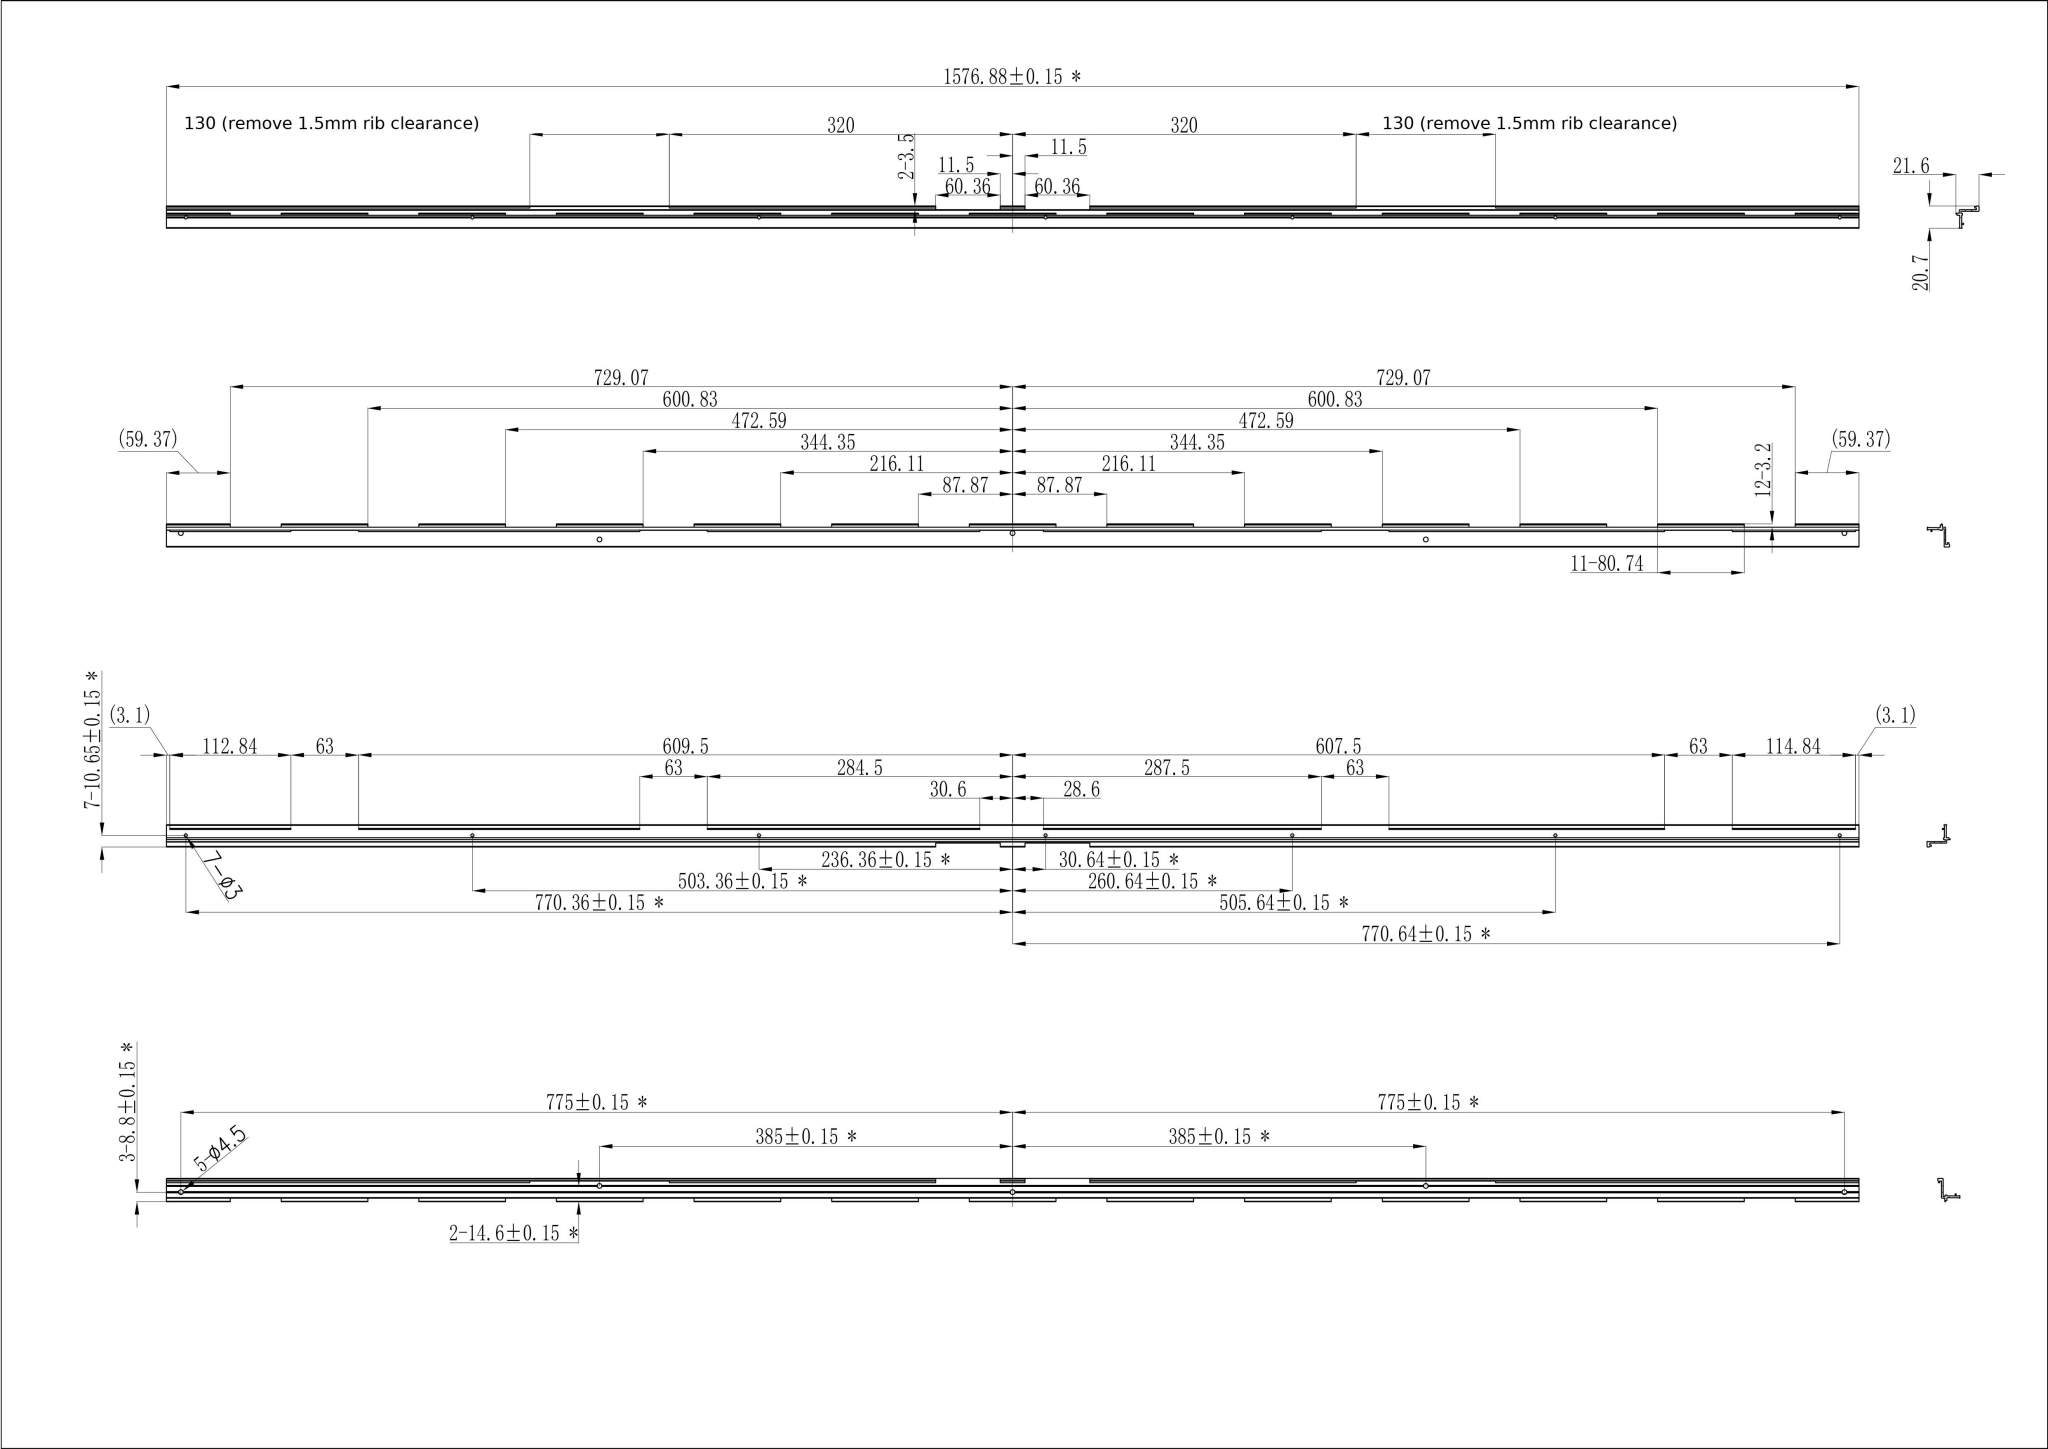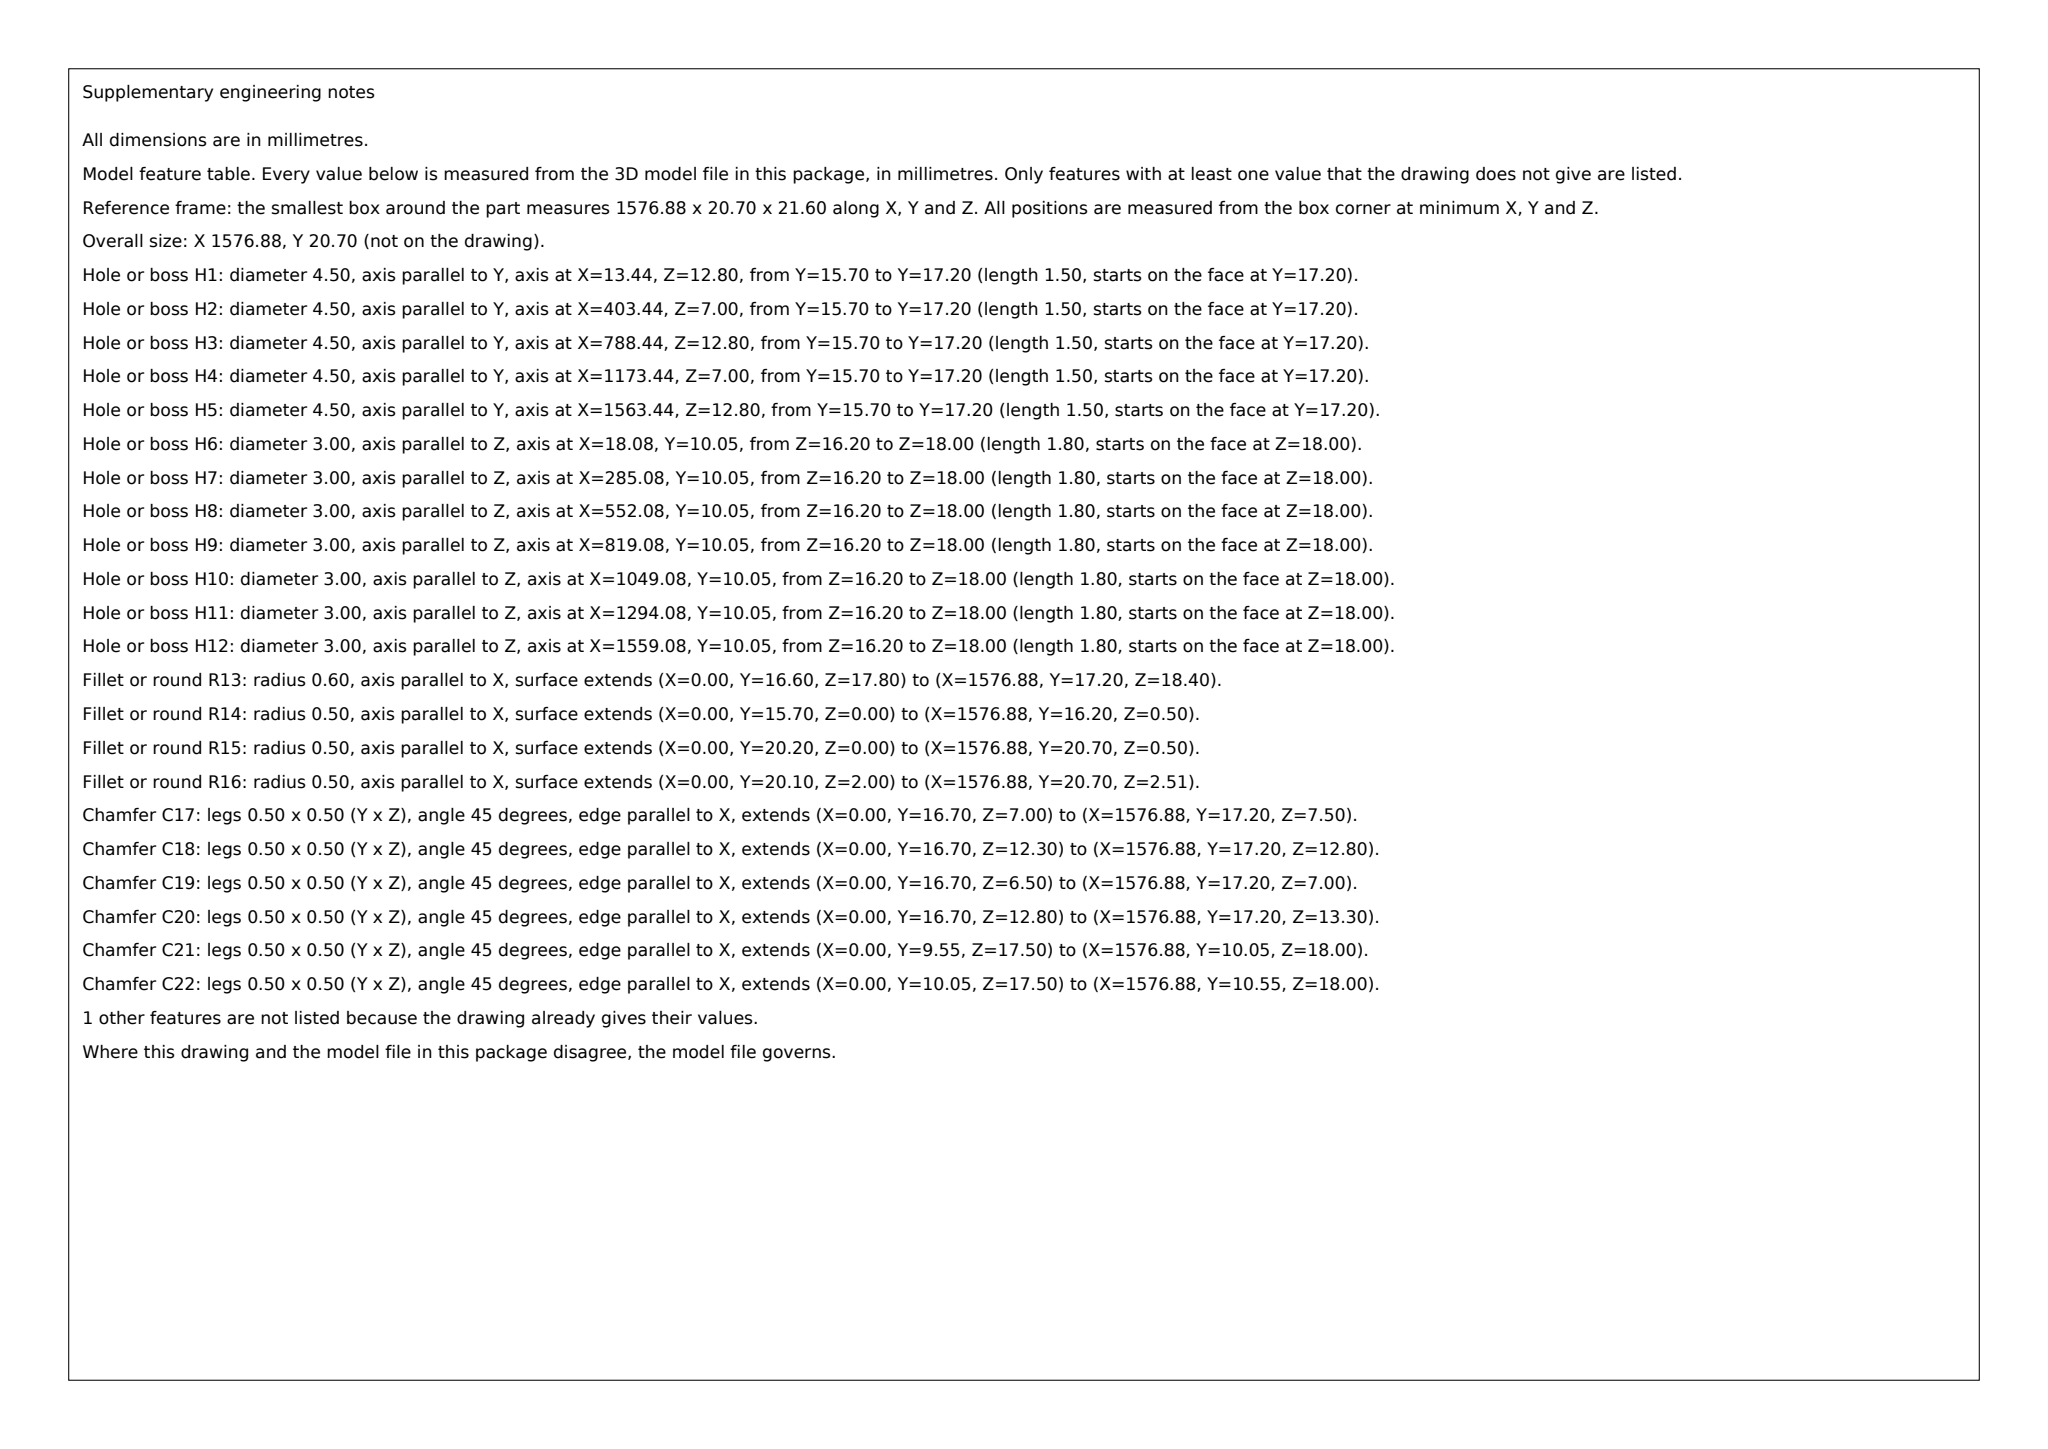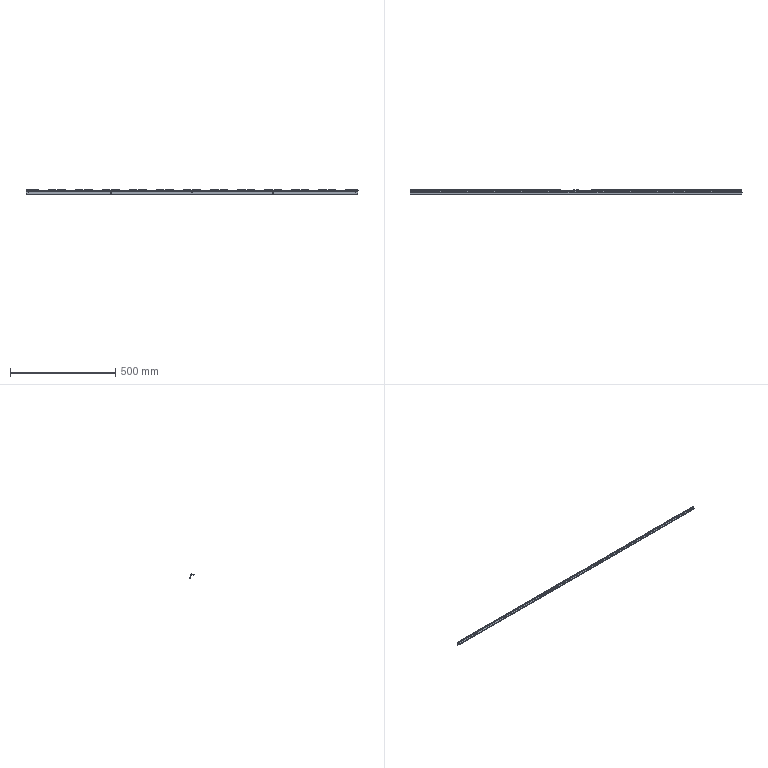Part | SolidWorks | mm | 1 solid | 236 faces | box 1576.88 x 20.7 x 21.6 mm | volume 111234 mm3 | plane 199 | cylinder 37 | commonest cylinder face diameters 3 x14 1 x12 4.5 x10 1.2 x1